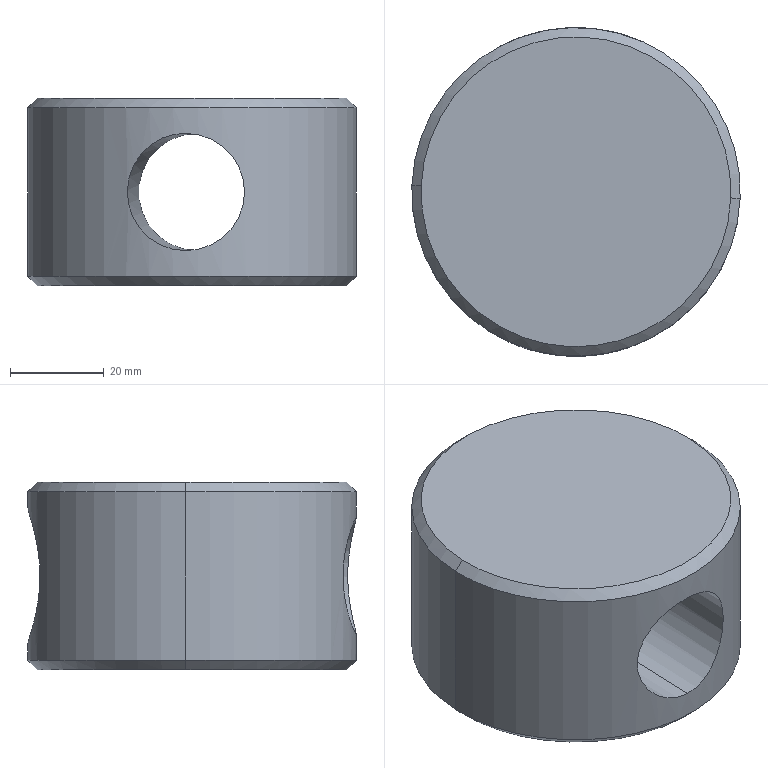Component | SolidWorks | Part3-1 | 1 solid | 13 faces | box 70 x 70 x 40 mm | volume 118313 mm3 | cylinder 6 | cone 4 | plane 3 | commonest cylinder face diameters 29 x2 25 x2 70 x2
build123d program:
from build123d import *

# Parameters (mm, degrees)
BOSS_EXTRUDE1_DEPTH   = 20
HOLE1_D               = 25
HOLE1_DEPTH           = 93.98
HOLE1_ON_FACE_2_D     = 25
HOLE1_ON_FACE_2_DEPTH = 93.98
HOLE2_D               = 29
HOLE2_DEPTH           = 7
CHAMFER1_SIZE         = 2


with BuildPart() as part:
    # Sketch1 → Boss-Extrude1 (new, symmetric)
    with BuildSketch(Plane.XY):
        with BuildLine():
            ThreePointArc((35, 0), (29.432, 18.941), (14.5, 31.855))
            Line((14.5, 31.855), (14.5, 24.855))
            Line((14.5, 24.855), (12.5, 24.855))
            Line((12.5, 24.855), (12.5, -32.692))
            ThreePointArc((12.5, -32.692), (28.831, -19.843), (35, 0))
        make_face()
        with BuildLine():
            Line((0, 24.855), (0, 35))
            ThreePointArc((0, 35), (-35, 0), (0, -35))
            Line((0, -35), (0, 24.855))
        make_face()
        with BuildLine():
            Line((12.5, 24.855), (0, 24.855))
            Line((0, 24.855), (0, -35))
            ThreePointArc((0, -35), (6.356, -34.418), (12.5, -32.692))
            Line((12.5, -32.692), (12.5, 24.855))
        make_face()
        with BuildLine():
            ThreePointArc((14.5, 31.855), (7.419, 34.205), (0, 35))
            Line((0, 35), (0, 24.855))
            Line((0, 24.855), (12.5, 24.855))
            Line((12.5, 24.855), (14.5, 24.855))
            Line((14.5, 24.855), (14.5, 31.855))
        make_face()
    extrude(amount=BOSS_EXTRUDE1_DEPTH, both=True)

    # Hole1
    with Locations(Plane(origin=(0, 35, 0), x_dir=(1, 0, 0), z_dir=(0, 1, 0))):
        with Locations((0, 0)):
            Hole(HOLE1_D / 2, depth=HOLE1_DEPTH)

    # Hole1 on face 2
    with Locations(Plane(origin=(0, 41.874, 0), x_dir=(1, 0, 0), z_dir=(0, 1, 0))):
        with Locations((0, 0)):
            Hole(HOLE1_ON_FACE_2_D / 2, depth=HOLE1_ON_FACE_2_DEPTH)

    # Hole2
    with Locations(Plane(origin=(0, 35, 0), x_dir=(1, 0, 0), z_dir=(0, 1, 0))):
        with Locations((0, 0)):
            Hole(HOLE2_D / 2, depth=HOLE2_DEPTH)

    # Chamfer1
    chamfer1_edges = [part.edges().sort_by_distance(p)[0] for p in [
        (29.432, 18.941, -20),
        (29.432, 18.941, 20),
    ]]
    chamfer(chamfer1_edges, length=CHAMFER1_SIZE)


solid = part.part

# Placed as in the assembly
solid = solid.moved(Location((-80.719, 26.515, 130), (0.000125, 0, -2.258)))
STEP:
#1=COLOUR_RGB('',0.7922,0.8196,0.9333);
#2=FILL_AREA_STYLE_COLOUR('',#1);
#3=FILL_AREA_STYLE('',(#2));
#4=SURFACE_STYLE_FILL_AREA(#3);
#5=SURFACE_SIDE_STYLE('',(#4));
#6=SURFACE_STYLE_USAGE(.BOTH.,#5);
#7=PRESENTATION_STYLE_ASSIGNMENT((#6));
#8=CARTESIAN_POINT('',(-1.88,0.9927,5.906));
#9=VERTEX_POINT('',#8);
#10=CARTESIAN_POINT('',(-4.476,1.095,5.906));
#11=VERTEX_POINT('',#10);
#12=CARTESIAN_POINT('',(-3.178,1.044,5.906));
#13=DIRECTION('',(0.,0.,1.));
#14=DIRECTION('',(0.9992,-0.03939,0.));
#15=AXIS2_PLACEMENT_3D('',#12,#13,#14);
#16=CIRCLE('',#15,1.299);
#17=EDGE_CURVE('',#9,#11,#16,.T.);
#18=ORIENTED_EDGE('',*,*,#17,.F.);
#19=CARTESIAN_POINT('',(-1.801,0.9896,5.827));
#20=VERTEX_POINT('',#19);
#21=CARTESIAN_POINT('',(-1.88,0.9927,5.906));
#22=DIRECTION('',(0.7066,-0.02785,-0.7071));
#23=VECTOR('',#22,39.37);
#24=LINE('',#21,#23);
#25=EDGE_CURVE('',#9,#20,#24,.T.);
#26=ORIENTED_EDGE('',*,*,#25,.T.);
#27=CARTESIAN_POINT('',(-4.555,1.098,5.827));
#28=VERTEX_POINT('',#27);
#29=CARTESIAN_POINT('',(-3.178,1.044,5.827));
#30=DIRECTION('',(-0.,-0.,-1.));
#31=DIRECTION('',(0.9992,-0.03939,0.));
#32=AXIS2_PLACEMENT_3D('',#29,#30,#31);
#33=CIRCLE('',#32,1.378);
#34=EDGE_CURVE('',#28,#20,#33,.T.);
#35=ORIENTED_EDGE('',*,*,#34,.F.);
#36=CARTESIAN_POINT('',(-4.476,1.095,5.906));
#37=DIRECTION('',(-0.7066,0.02785,-0.7071));
#38=VECTOR('',#37,39.37);
#39=LINE('',#36,#38);
#40=EDGE_CURVE('',#11,#28,#39,.T.);
#41=ORIENTED_EDGE('',*,*,#40,.F.);
#42=EDGE_LOOP('',(#18,#26,#35,#41));
#43=FACE_OUTER_BOUND('',#42,.T.);
#44=CARTESIAN_POINT('',(-3.178,1.044,5.906));
#45=DIRECTION('',(-0.,-0.,-1.));
#46=DIRECTION('',(-0.9992,0.03939,0.));
#47=AXIS2_PLACEMENT_3D('',#44,#45,#46);
#48=CONICAL_SURFACE('',#47,1.299,0.7854);
#49=ADVANCED_FACE('',(#43),#48,.T.);
#50=CARTESIAN_POINT('',(-4.476,1.095,4.331));
#51=VERTEX_POINT('',#50);
#52=CARTESIAN_POINT('',(-1.88,0.9927,4.331));
#53=VERTEX_POINT('',#52);
#54=CARTESIAN_POINT('',(-3.178,1.044,4.331));
#55=DIRECTION('',(-0.,-0.,-1.));
#56=DIRECTION('',(0.9992,-0.03939,0.));
#57=AXIS2_PLACEMENT_3D('',#54,#55,#56);
#58=CIRCLE('',#57,1.299);
#59=EDGE_CURVE('',#51,#53,#58,.T.);
#60=ORIENTED_EDGE('',*,*,#59,.F.);
#61=CARTESIAN_POINT('',(-4.555,1.098,4.409));
#62=VERTEX_POINT('',#61);
#63=CARTESIAN_POINT('',(-4.555,1.098,4.409));
#64=DIRECTION('',(-0.7066,0.02785,0.7071));
#65=VECTOR('',#64,39.37);
#66=LINE('',#63,#65);
#67=EDGE_CURVE('',#51,#62,#66,.T.);
#68=ORIENTED_EDGE('',*,*,#67,.T.);
#69=CARTESIAN_POINT('',(-1.801,0.9896,4.409));
#70=VERTEX_POINT('',#69);
#71=CARTESIAN_POINT('',(-3.178,1.044,4.409));
#72=DIRECTION('',(0.,0.,1.));
#73=DIRECTION('',(0.9992,-0.03939,0.));
#74=AXIS2_PLACEMENT_3D('',#71,#72,#73);
#75=CIRCLE('',#74,1.378);
#76=EDGE_CURVE('',#70,#62,#75,.T.);
#77=ORIENTED_EDGE('',*,*,#76,.F.);
#78=CARTESIAN_POINT('',(-1.801,0.9896,4.409));
#79=DIRECTION('',(0.7066,-0.02785,0.7071));
#80=VECTOR('',#79,39.37);
#81=LINE('',#78,#80);
#82=EDGE_CURVE('',#53,#70,#81,.T.);
#83=ORIENTED_EDGE('',*,*,#82,.F.);
#84=EDGE_LOOP('',(#60,#68,#77,#83));
#85=FACE_OUTER_BOUND('',#84,.T.);
#86=CARTESIAN_POINT('',(-3.178,1.044,4.409));
#87=DIRECTION('',(0.,0.,1.));
#88=DIRECTION('',(0.9992,-0.03939,0.));
#89=AXIS2_PLACEMENT_3D('',#86,#87,#88);
#90=CONICAL_SURFACE('',#89,1.378,0.7854);
#91=ADVANCED_FACE('',(#85),#90,.T.);
#92=CARTESIAN_POINT('',(-3.134,2.145,4.547));
#93=VERTEX_POINT('',#92);
#94=CARTESIAN_POINT('',(-3.134,2.145,5.689));
#95=VERTEX_POINT('',#94);
#96=CARTESIAN_POINT('',(-3.134,2.145,5.118));
#97=DIRECTION('',(0.03939,0.9992,-0.));
#98=DIRECTION('',(0.,0.,1.));
#99=AXIS2_PLACEMENT_3D('',#96,#97,#98);
#100=CIRCLE('',#99,0.5709);
#101=EDGE_CURVE('',#93,#95,#100,.T.);
#102=ORIENTED_EDGE('',*,*,#101,.F.);
#103=CARTESIAN_POINT('',(-3.124,2.421,4.547));
#104=VERTEX_POINT('',#103);
#105=CARTESIAN_POINT('',(-3.124,2.421,4.547));
#106=DIRECTION('',(0.03939,0.9992,-0.));
#107=VECTOR('',#106,39.37);
#108=LINE('',#105,#107);
#109=EDGE_CURVE('',#93,#104,#108,.T.);
#110=ORIENTED_EDGE('',*,*,#109,.T.);
#111=CARTESIAN_POINT('',(-3.124,2.421,5.689));
#112=VERTEX_POINT('',#111);
#113=CARTESIAN_POINT('',(-3.124,2.421,5.689));
#114=CARTESIAN_POINT('',(-3.162,2.422,5.689));
#115=CARTESIAN_POINT('',(-3.199,2.422,5.685));
#116=CARTESIAN_POINT('',(-3.255,2.42,5.674));
#117=CARTESIAN_POINT('',(-3.273,2.419,5.669));
#118=CARTESIAN_POINT('',(-3.309,2.416,5.658));
#119=CARTESIAN_POINT('',(-3.327,2.414,5.652));
#120=CARTESIAN_POINT('',(-3.379,2.408,5.63));
#121=CARTESIAN_POINT('',(-3.412,2.402,5.613));
#122=CARTESIAN_POINT('',(-3.459,2.393,5.582));
#123=CARTESIAN_POINT('',(-3.474,2.39,5.57));
#124=CARTESIAN_POINT('',(-3.503,2.383,5.547));
#125=CARTESIAN_POINT('',(-3.516,2.38,5.535));
#126=CARTESIAN_POINT('',(-3.543,2.373,5.508));
#127=CARTESIAN_POINT('',(-3.555,2.369,5.495));
#128=CARTESIAN_POINT('',(-3.579,2.362,5.466));
#129=CARTESIAN_POINT('',(-3.59,2.359,5.451));
#130=CARTESIAN_POINT('',(-3.622,2.349,5.405));
#131=CARTESIAN_POINT('',(-3.64,2.342,5.372));
#132=CARTESIAN_POINT('',(-3.661,2.334,5.321));
#133=CARTESIAN_POINT('',(-3.668,2.332,5.303));
#134=CARTESIAN_POINT('',(-3.679,2.327,5.267));
#135=CARTESIAN_POINT('',(-3.684,2.326,5.249));
#136=CARTESIAN_POINT('',(-3.695,2.321,5.194));
#137=CARTESIAN_POINT('',(-3.699,2.32,5.156));
#138=CARTESIAN_POINT('',(-3.699,2.32,5.1));
#139=CARTESIAN_POINT('',(-3.698,2.32,5.081));
#140=CARTESIAN_POINT('',(-3.694,2.321,5.043));
#141=CARTESIAN_POINT('',(-3.691,2.323,5.024));
#142=CARTESIAN_POINT('',(-3.684,2.326,4.987));
#143=CARTESIAN_POINT('',(-3.679,2.327,4.969));
#144=CARTESIAN_POINT('',(-3.668,2.332,4.933));
#145=CARTESIAN_POINT('',(-3.662,2.334,4.916));
#146=CARTESIAN_POINT('',(-3.639,2.342,4.863));
#147=CARTESIAN_POINT('',(-3.622,2.349,4.831));
#148=CARTESIAN_POINT('',(-3.59,2.359,4.785));
#149=CARTESIAN_POINT('',(-3.579,2.362,4.77));
#150=CARTESIAN_POINT('',(-3.555,2.369,4.741));
#151=CARTESIAN_POINT('',(-3.542,2.373,4.727));
#152=CARTESIAN_POINT('',(-3.503,2.383,4.688));
#153=CARTESIAN_POINT('',(-3.474,2.39,4.665));
#154=CARTESIAN_POINT('',(-3.427,2.399,4.634));
#155=CARTESIAN_POINT('',(-3.411,2.402,4.624));
#156=CARTESIAN_POINT('',(-3.378,2.407,4.606));
#157=CARTESIAN_POINT('',(-3.361,2.41,4.598));
#158=CARTESIAN_POINT('',(-3.309,2.416,4.577));
#159=CARTESIAN_POINT('',(-3.274,2.419,4.566));
#160=CARTESIAN_POINT('',(-3.218,2.421,4.555));
#161=CARTESIAN_POINT('',(-3.199,2.422,4.552));
#162=CARTESIAN_POINT('',(-3.161,2.422,4.548));
#163=CARTESIAN_POINT('',(-3.142,2.422,4.547));
#164=CARTESIAN_POINT('',(-3.124,2.421,4.547));
#165=B_SPLINE_CURVE_WITH_KNOTS('',3,(#113,#114,#115,#116,#117,#118,#119,#120,#121,#122,#123,#124,#125,#126,#127,#128,#129,#130,#131,#132,#133,#134,#135,#136,#137,#138,#139,#140,#141,#142,#143,#144,#145,#146,#147,#148,#149,#150,#151,#152,#153,#154,#155,#156,#157,#158,#159,#160,#161,#162,#163,#164),.UNSPECIFIED.,.F.,.F.,(4,2,2,2,2,2,2,2,2,2,2,2,2,2,2,2,2,2,2,2,2,2,2,2,2,4),(0.,0.002866,0.004299,0.005732,0.008598,0.01003,0.01146,0.0129,0.01433,0.0172,0.01863,0.02006,0.02293,0.02436,0.02579,0.02723,0.02866,0.03153,0.03296,0.03439,0.03726,0.03869,0.04012,0.04299,0.04442,0.04586),.UNSPECIFIED.);
#166=EDGE_CURVE('',#112,#104,#165,.T.);
#167=ORIENTED_EDGE('',*,*,#166,.F.);
#168=CARTESIAN_POINT('',(-3.124,2.421,5.689));
#169=DIRECTION('',(0.03939,0.9992,-0.));
#170=VECTOR('',#169,39.37);
#171=LINE('',#168,#170);
#172=EDGE_CURVE('',#95,#112,#171,.T.);
#173=ORIENTED_EDGE('',*,*,#172,.F.);
#174=EDGE_LOOP('',(#102,#110,#167,#173));
#175=FACE_OUTER_BOUND('',#174,.T.);
#176=CARTESIAN_POINT('',(-3.124,2.421,5.118));
#177=DIRECTION('',(0.03939,0.9992,-0.));
#178=DIRECTION('',(0.,0.,1.));
#179=AXIS2_PLACEMENT_3D('',#176,#177,#178);
#180=CYLINDRICAL_SURFACE('',#179,0.5709);
#181=ADVANCED_FACE('',(#175),#180,.F.);
#182=CARTESIAN_POINT('',(-3.232,-0.333,4.626));
#183=VERTEX_POINT('',#182);
#184=CARTESIAN_POINT('',(-3.232,-0.333,5.61));
#185=VERTEX_POINT('',#184);
#186=CARTESIAN_POINT('',(-3.232,-0.333,4.626));
#187=CARTESIAN_POINT('',(-3.248,-0.3324,4.626));
#188=CARTESIAN_POINT('',(-3.264,-0.3314,4.627));
#189=CARTESIAN_POINT('',(-3.297,-0.329,4.63));
#190=CARTESIAN_POINT('',(-3.313,-0.3275,4.632));
#191=CARTESIAN_POINT('',(-3.361,-0.3223,4.642));
#192=CARTESIAN_POINT('',(-3.391,-0.3178,4.651));
#193=CARTESIAN_POINT('',(-3.436,-0.3099,4.67));
#194=CARTESIAN_POINT('',(-3.45,-0.307,4.677));
#195=CARTESIAN_POINT('',(-3.478,-0.301,4.692));
#196=CARTESIAN_POINT('',(-3.492,-0.2979,4.701));
#197=CARTESIAN_POINT('',(-3.531,-0.2882,4.727));
#198=CARTESIAN_POINT('',(-3.556,-0.2814,4.748));
#199=CARTESIAN_POINT('',(-3.59,-0.2712,4.782));
#200=CARTESIAN_POINT('',(-3.6,-0.2678,4.794));
#201=CARTESIAN_POINT('',(-3.62,-0.2612,4.818));
#202=CARTESIAN_POINT('',(-3.63,-0.258,4.831));
#203=CARTESIAN_POINT('',(-3.647,-0.2518,4.858));
#204=CARTESIAN_POINT('',(-3.655,-0.2488,4.871));
#205=CARTESIAN_POINT('',(-3.67,-0.2432,4.899));
#206=CARTESIAN_POINT('',(-3.677,-0.2405,4.914));
#207=CARTESIAN_POINT('',(-3.695,-0.2333,4.959));
#208=CARTESIAN_POINT('',(-3.705,-0.2294,4.99));
#209=CARTESIAN_POINT('',(-3.714,-0.2255,5.037));
#210=CARTESIAN_POINT('',(-3.716,-0.2245,5.053));
#211=CARTESIAN_POINT('',(-3.72,-0.2231,5.086));
#212=CARTESIAN_POINT('',(-3.72,-0.2228,5.102));
#213=CARTESIAN_POINT('',(-3.72,-0.2228,5.151));
#214=CARTESIAN_POINT('',(-3.717,-0.2242,5.183));
#215=CARTESIAN_POINT('',(-3.708,-0.2281,5.231));
#216=CARTESIAN_POINT('',(-3.704,-0.2298,5.247));
#217=CARTESIAN_POINT('',(-3.695,-0.2336,5.277));
#218=CARTESIAN_POINT('',(-3.689,-0.2357,5.293));
#219=CARTESIAN_POINT('',(-3.677,-0.2405,5.322));
#220=CARTESIAN_POINT('',(-3.67,-0.2432,5.337));
#221=CARTESIAN_POINT('',(-3.655,-0.2488,5.365));
#222=CARTESIAN_POINT('',(-3.647,-0.2518,5.379));
#223=CARTESIAN_POINT('',(-3.62,-0.2612,5.419));
#224=CARTESIAN_POINT('',(-3.6,-0.2679,5.444));
#225=CARTESIAN_POINT('',(-3.556,-0.2814,5.489));
#226=CARTESIAN_POINT('',(-3.531,-0.2883,5.509));
#227=CARTESIAN_POINT('',(-3.478,-0.3012,5.545));
#228=CARTESIAN_POINT('',(-3.45,-0.3072,5.56));
#229=CARTESIAN_POINT('',(-3.406,-0.3151,5.579));
#230=CARTESIAN_POINT('',(-3.391,-0.3176,5.584));
#231=CARTESIAN_POINT('',(-3.36,-0.3221,5.594));
#232=CARTESIAN_POINT('',(-3.344,-0.3241,5.598));
#233=CARTESIAN_POINT('',(-3.297,-0.3293,5.607));
#234=CARTESIAN_POINT('',(-3.265,-0.3317,5.61));
#235=CARTESIAN_POINT('',(-3.232,-0.333,5.61));
#236=B_SPLINE_CURVE_WITH_KNOTS('',3,(#186,#187,#188,#189,#190,#191,#192,#193,#194,#195,#196,#197,#198,#199,#200,#201,#202,#203,#204,#205,#206,#207,#208,#209,#210,#211,#212,#213,#214,#215,#216,#217,#218,#219,#220,#221,#222,#223,#224,#225,#226,#227,#228,#229,#230,#231,#232,#233,#234,#235),.UNSPECIFIED.,.F.,.F.,(4,2,2,2,2,2,2,2,2,2,2,2,2,2,2,2,2,2,2,2,2,2,2,2,4),(0.03941,0.04064,0.04187,0.04433,0.04557,0.0468,0.04926,0.05049,0.05172,0.05295,0.05418,0.05665,0.05788,0.05911,0.06157,0.0628,0.06403,0.06526,0.0665,0.06896,0.07142,0.07388,0.07511,0.07635,0.07881),.UNSPECIFIED.);
#237=EDGE_CURVE('',#183,#185,#236,.T.);
#238=ORIENTED_EDGE('',*,*,#237,.F.);
#239=CARTESIAN_POINT('',(-3.134,2.145,4.626));
#240=VERTEX_POINT('',#239);
#241=CARTESIAN_POINT('',(-3.124,2.421,4.626));
#242=DIRECTION('',(0.03939,0.9992,-0.));
#243=VECTOR('',#242,39.37);
#244=LINE('',#241,#243);
#245=EDGE_CURVE('',#183,#240,#244,.T.);
#246=ORIENTED_EDGE('',*,*,#245,.T.);
#247=CARTESIAN_POINT('',(-3.134,2.145,5.61));
#248=VERTEX_POINT('',#247);
#249=CARTESIAN_POINT('',(-3.134,2.145,5.118));
#250=DIRECTION('',(0.03939,0.9992,-0.));
#251=DIRECTION('',(-0.,0.,-1.));
#252=AXIS2_PLACEMENT_3D('',#249,#250,#251);
#253=CIRCLE('',#252,0.4921);
#254=EDGE_CURVE('',#240,#248,#253,.T.);
#255=ORIENTED_EDGE('',*,*,#254,.T.);
#256=CARTESIAN_POINT('',(-3.124,2.421,5.61));
#257=DIRECTION('',(0.03939,0.9992,-0.));
#258=VECTOR('',#257,39.37);
#259=LINE('',#256,#258);
#260=EDGE_CURVE('',#185,#248,#259,.T.);
#261=ORIENTED_EDGE('',*,*,#260,.F.);
#262=EDGE_LOOP('',(#238,#246,#255,#261));
#263=FACE_OUTER_BOUND('',#262,.T.);
#264=CARTESIAN_POINT('',(-3.124,2.421,5.118));
#265=DIRECTION('',(0.03939,0.9992,-0.));
#266=DIRECTION('',(0.,0.,1.));
#267=AXIS2_PLACEMENT_3D('',#264,#265,#266);
#268=CYLINDRICAL_SURFACE('',#267,0.4921);
#269=ADVANCED_FACE('',(#263),#268,.F.);
#270=ORIENTED_EDGE('',*,*,#166,.T.);
#271=CARTESIAN_POINT('',(-3.124,2.421,4.547));
#272=CARTESIAN_POINT('',(-3.105,2.42,4.547));
#273=CARTESIAN_POINT('',(-3.086,2.419,4.548));
#274=CARTESIAN_POINT('',(-3.048,2.416,4.552));
#275=CARTESIAN_POINT('',(-3.03,2.414,4.555));
#276=CARTESIAN_POINT('',(-2.974,2.407,4.566));
#277=CARTESIAN_POINT('',(-2.939,2.401,4.577));
#278=CARTESIAN_POINT('',(-2.887,2.391,4.599));
#279=CARTESIAN_POINT('',(-2.87,2.387,4.607));
#280=CARTESIAN_POINT('',(-2.838,2.379,4.624));
#281=CARTESIAN_POINT('',(-2.822,2.375,4.634));
#282=CARTESIAN_POINT('',(-2.792,2.367,4.655));
#283=CARTESIAN_POINT('',(-2.777,2.362,4.666));
#284=CARTESIAN_POINT('',(-2.749,2.353,4.689));
#285=CARTESIAN_POINT('',(-2.735,2.349,4.702));
#286=CARTESIAN_POINT('',(-2.696,2.335,4.741));
#287=CARTESIAN_POINT('',(-2.673,2.326,4.77));
#288=CARTESIAN_POINT('',(-2.643,2.314,4.815));
#289=CARTESIAN_POINT('',(-2.634,2.31,4.831));
#290=CARTESIAN_POINT('',(-2.616,2.302,4.864));
#291=CARTESIAN_POINT('',(-2.608,2.299,4.881));
#292=CARTESIAN_POINT('',(-2.587,2.289,4.933));
#293=CARTESIAN_POINT('',(-2.576,2.284,4.968));
#294=CARTESIAN_POINT('',(-2.566,2.278,5.024));
#295=CARTESIAN_POINT('',(-2.563,2.277,5.042));
#296=CARTESIAN_POINT('',(-2.559,2.275,5.08));
#297=CARTESIAN_POINT('',(-2.558,2.275,5.099));
#298=CARTESIAN_POINT('',(-2.558,2.275,5.156));
#299=CARTESIAN_POINT('',(-2.562,2.276,5.193));
#300=CARTESIAN_POINT('',(-2.576,2.284,5.268));
#301=CARTESIAN_POINT('',(-2.587,2.289,5.303));
#302=CARTESIAN_POINT('',(-2.608,2.299,5.355));
#303=CARTESIAN_POINT('',(-2.616,2.302,5.372));
#304=CARTESIAN_POINT('',(-2.634,2.31,5.405));
#305=CARTESIAN_POINT('',(-2.643,2.314,5.421));
#306=CARTESIAN_POINT('',(-2.674,2.326,5.467));
#307=CARTESIAN_POINT('',(-2.697,2.335,5.495));
#308=CARTESIAN_POINT('',(-2.735,2.349,5.535));
#309=CARTESIAN_POINT('',(-2.749,2.353,5.547));
#310=CARTESIAN_POINT('',(-2.777,2.362,5.571));
#311=CARTESIAN_POINT('',(-2.792,2.367,5.582));
#312=CARTESIAN_POINT('',(-2.837,2.379,5.613));
#313=CARTESIAN_POINT('',(-2.87,2.387,5.63));
#314=CARTESIAN_POINT('',(-2.939,2.401,5.659));
#315=CARTESIAN_POINT('',(-2.975,2.407,5.67));
#316=CARTESIAN_POINT('',(-3.029,2.414,5.681));
#317=CARTESIAN_POINT('',(-3.048,2.416,5.684));
#318=CARTESIAN_POINT('',(-3.085,2.419,5.688));
#319=CARTESIAN_POINT('',(-3.105,2.42,5.689));
#320=CARTESIAN_POINT('',(-3.124,2.421,5.689));
#321=B_SPLINE_CURVE_WITH_KNOTS('',3,(#271,#272,#273,#274,#275,#276,#277,#278,#279,#280,#281,#282,#283,#284,#285,#286,#287,#288,#289,#290,#291,#292,#293,#294,#295,#296,#297,#298,#299,#300,#301,#302,#303,#304,#305,#306,#307,#308,#309,#310,#311,#312,#313,#314,#315,#316,#317,#318,#319,#320),.UNSPECIFIED.,.F.,.F.,(4,2,2,2,2,2,2,2,2,2,2,2,2,2,2,2,2,2,2,2,2,2,2,2,4),(0.04586,0.04729,0.04872,0.05158,0.05302,0.05445,0.05588,0.05731,0.06018,0.06161,0.06304,0.0659,0.06733,0.06877,0.07163,0.07449,0.07593,0.07736,0.08022,0.08165,0.08309,0.08595,0.08881,0.09025,0.09168),.UNSPECIFIED.);
#322=EDGE_CURVE('',#104,#112,#321,.T.);
#323=ORIENTED_EDGE('',*,*,#322,.T.);
#324=EDGE_LOOP('',(#270,#323));
#325=FACE_BOUND('',#324,.T.);
#326=ORIENTED_EDGE('',*,*,#34,.T.);
#327=CARTESIAN_POINT('',(-1.801,0.9896,5.906));
#328=DIRECTION('',(-0.,-0.,-1.));
#329=VECTOR('',#328,39.37);
#330=LINE('',#327,#329);
#331=EDGE_CURVE('',#20,#70,#330,.T.);
#332=ORIENTED_EDGE('',*,*,#331,.T.);
#333=ORIENTED_EDGE('',*,*,#76,.T.);
#334=CARTESIAN_POINT('',(-4.555,1.098,5.906));
#335=DIRECTION('',(-0.,-0.,-1.));
#336=VECTOR('',#335,39.37);
#337=LINE('',#334,#336);
#338=EDGE_CURVE('',#28,#62,#337,.T.);
#339=ORIENTED_EDGE('',*,*,#338,.F.);
#340=EDGE_LOOP('',(#326,#332,#333,#339));
#341=FACE_OUTER_BOUND('',#340,.T.);
#342=CARTESIAN_POINT('',(-3.178,1.044,5.906));
#343=DIRECTION('',(-0.,-0.,-1.));
#344=DIRECTION('',(-0.9992,0.03939,0.));
#345=AXIS2_PLACEMENT_3D('',#342,#343,#344);
#346=CYLINDRICAL_SURFACE('',#345,1.378);
#347=ADVANCED_FACE('',(#325,#341),#346,.T.);
#348=ORIENTED_EDGE('',*,*,#331,.F.);
#349=CARTESIAN_POINT('',(-3.178,1.044,5.827));
#350=DIRECTION('',(-0.,-0.,-1.));
#351=DIRECTION('',(0.9992,-0.03939,0.));
#352=AXIS2_PLACEMENT_3D('',#349,#350,#351);
#353=CIRCLE('',#352,1.378);
#354=EDGE_CURVE('',#20,#28,#353,.T.);
#355=ORIENTED_EDGE('',*,*,#354,.T.);
#356=ORIENTED_EDGE('',*,*,#338,.T.);
#357=CARTESIAN_POINT('',(-3.178,1.044,4.409));
#358=DIRECTION('',(0.,0.,1.));
#359=DIRECTION('',(0.9992,-0.03939,0.));
#360=AXIS2_PLACEMENT_3D('',#357,#358,#359);
#361=CIRCLE('',#360,1.378);
#362=EDGE_CURVE('',#62,#70,#361,.T.);
#363=ORIENTED_EDGE('',*,*,#362,.T.);
#364=EDGE_LOOP('',(#348,#355,#356,#363));
#365=FACE_OUTER_BOUND('',#364,.T.);
#366=CARTESIAN_POINT('',(-3.232,-0.333,5.61));
#367=CARTESIAN_POINT('',(-3.199,-0.3343,5.61));
#368=CARTESIAN_POINT('',(-3.167,-0.3344,5.607));
#369=CARTESIAN_POINT('',(-3.12,-0.3329,5.597));
#370=CARTESIAN_POINT('',(-3.104,-0.3322,5.594));
#371=CARTESIAN_POINT('',(-3.073,-0.3301,5.584));
#372=CARTESIAN_POINT('',(-3.057,-0.3289,5.579));
#373=CARTESIAN_POINT('',(-3.012,-0.3244,5.56));
#374=CARTESIAN_POINT('',(-2.984,-0.3206,5.545));
#375=CARTESIAN_POINT('',(-2.944,-0.3141,5.518));
#376=CARTESIAN_POINT('',(-2.931,-0.3118,5.508));
#377=CARTESIAN_POINT('',(-2.906,-0.307,5.488));
#378=CARTESIAN_POINT('',(-2.894,-0.3045,5.477));
#379=CARTESIAN_POINT('',(-2.86,-0.2971,5.443));
#380=CARTESIAN_POINT('',(-2.839,-0.292,5.419));
#381=CARTESIAN_POINT('',(-2.803,-0.2822,5.365));
#382=CARTESIAN_POINT('',(-2.788,-0.2777,5.337));
#383=CARTESIAN_POINT('',(-2.769,-0.272,5.293));
#384=CARTESIAN_POINT('',(-2.763,-0.2703,5.277));
#385=CARTESIAN_POINT('',(-2.754,-0.2672,5.247));
#386=CARTESIAN_POINT('',(-2.75,-0.2659,5.231));
#387=CARTESIAN_POINT('',(-2.74,-0.2627,5.183));
#388=CARTESIAN_POINT('',(-2.737,-0.2616,5.151));
#389=CARTESIAN_POINT('',(-2.737,-0.2616,5.102));
#390=CARTESIAN_POINT('',(-2.738,-0.2618,5.086));
#391=CARTESIAN_POINT('',(-2.741,-0.2629,5.053));
#392=CARTESIAN_POINT('',(-2.743,-0.2638,5.037));
#393=CARTESIAN_POINT('',(-2.753,-0.2669,4.99));
#394=CARTESIAN_POINT('',(-2.763,-0.27,4.959));
#395=CARTESIAN_POINT('',(-2.788,-0.2778,4.899));
#396=CARTESIAN_POINT('',(-2.803,-0.2823,4.871));
#397=CARTESIAN_POINT('',(-2.83,-0.2895,4.831));
#398=CARTESIAN_POINT('',(-2.84,-0.292,4.818));
#399=CARTESIAN_POINT('',(-2.86,-0.297,4.793));
#400=CARTESIAN_POINT('',(-2.871,-0.2996,4.781));
#401=CARTESIAN_POINT('',(-2.906,-0.3071,4.747));
#402=CARTESIAN_POINT('',(-2.93,-0.3119,4.727));
#403=CARTESIAN_POINT('',(-2.971,-0.3185,4.7));
#404=CARTESIAN_POINT('',(-2.985,-0.3205,4.692));
#405=CARTESIAN_POINT('',(-3.013,-0.3243,4.677));
#406=CARTESIAN_POINT('',(-3.028,-0.326,4.67));
#407=CARTESIAN_POINT('',(-3.072,-0.3304,4.651));
#408=CARTESIAN_POINT('',(-3.103,-0.3324,4.642));
#409=CARTESIAN_POINT('',(-3.151,-0.3339,4.632));
#410=CARTESIAN_POINT('',(-3.168,-0.3341,4.63));
#411=CARTESIAN_POINT('',(-3.2,-0.334,4.627));
#412=CARTESIAN_POINT('',(-3.216,-0.3336,4.626));
#413=CARTESIAN_POINT('',(-3.232,-0.333,4.626));
#414=B_SPLINE_CURVE_WITH_KNOTS('',3,(#366,#367,#368,#369,#370,#371,#372,#373,#374,#375,#376,#377,#378,#379,#380,#381,#382,#383,#384,#385,#386,#387,#388,#389,#390,#391,#392,#393,#394,#395,#396,#397,#398,#399,#400,#401,#402,#403,#404,#405,#406,#407,#408,#409,#410,#411,#412,#413),.UNSPECIFIED.,.F.,.F.,(4,2,2,2,2,2,2,2,2,2,2,2,2,2,2,2,2,2,2,2,2,2,2,4),(0.,0.002463,0.003695,0.004926,0.007389,0.008621,0.009852,0.01232,0.01478,0.01601,0.01724,0.0197,0.02094,0.02217,0.02463,0.02709,0.02833,0.02956,0.03202,0.03325,0.03448,0.03695,0.03818,0.03941),.UNSPECIFIED.);
#415=EDGE_CURVE('',#185,#183,#414,.T.);
#416=ORIENTED_EDGE('',*,*,#415,.T.);
#417=ORIENTED_EDGE('',*,*,#237,.T.);
#418=EDGE_LOOP('',(#416,#417));
#419=FACE_BOUND('',#418,.T.);
#420=CARTESIAN_POINT('',(-3.178,1.044,5.906));
#421=DIRECTION('',(-0.,-0.,-1.));
#422=DIRECTION('',(-0.9992,0.03939,0.));
#423=AXIS2_PLACEMENT_3D('',#420,#421,#422);
#424=CYLINDRICAL_SURFACE('',#423,1.378);
#425=ADVANCED_FACE('',(#365,#419),#424,.T.);
#426=CARTESIAN_POINT('',(-3.178,1.044,5.906));
#427=DIRECTION('',(0.,0.,1.));
#428=DIRECTION('',(0.9992,-0.03939,0.));
#429=AXIS2_PLACEMENT_3D('',#426,#427,#428);
#430=CIRCLE('',#429,1.299);
#431=EDGE_CURVE('',#11,#9,#430,.T.);
#432=ORIENTED_EDGE('',*,*,#431,.T.);
#433=ORIENTED_EDGE('',*,*,#17,.T.);
#434=EDGE_LOOP('',(#432,#433));
#435=FACE_OUTER_BOUND('',#434,.T.);
#436=CARTESIAN_POINT('',(-3.178,1.044,5.906));
#437=DIRECTION('',(0.,0.,1.));
#438=DIRECTION('',(0.9992,-0.03939,-0.));
#439=AXIS2_PLACEMENT_3D('',#436,#437,#438);
#440=PLANE('',#439);
#441=ADVANCED_FACE('',(#435),#440,.T.);
#442=CARTESIAN_POINT('',(-3.178,1.044,4.331));
#443=DIRECTION('',(-0.,-0.,-1.));
#444=DIRECTION('',(0.9992,-0.03939,0.));
#445=AXIS2_PLACEMENT_3D('',#442,#443,#444);
#446=CIRCLE('',#445,1.299);
#447=EDGE_CURVE('',#53,#51,#446,.T.);
#448=ORIENTED_EDGE('',*,*,#447,.T.);
#449=ORIENTED_EDGE('',*,*,#59,.T.);
#450=EDGE_LOOP('',(#448,#449));
#451=FACE_OUTER_BOUND('',#450,.T.);
#452=CARTESIAN_POINT('',(-3.178,1.044,4.331));
#453=DIRECTION('',(0.,0.,1.));
#454=DIRECTION('',(0.9992,-0.03939,-0.));
#455=AXIS2_PLACEMENT_3D('',#452,#453,#454);
#456=PLANE('',#455);
#457=ADVANCED_FACE('',(#451),#456,.F.);
#458=ORIENTED_EDGE('',*,*,#245,.F.);
#459=ORIENTED_EDGE('',*,*,#415,.F.);
#460=ORIENTED_EDGE('',*,*,#260,.T.);
#461=CARTESIAN_POINT('',(-3.134,2.145,5.118));
#462=DIRECTION('',(0.03939,0.9992,-0.));
#463=DIRECTION('',(0.,0.,-1.));
#464=AXIS2_PLACEMENT_3D('',#461,#462,#463);
#465=CIRCLE('',#464,0.4921);
#466=EDGE_CURVE('',#248,#240,#465,.T.);
#467=ORIENTED_EDGE('',*,*,#466,.T.);
#468=EDGE_LOOP('',(#458,#459,#460,#467));
#469=FACE_OUTER_BOUND('',#468,.T.);
#470=CARTESIAN_POINT('',(-3.124,2.421,5.118));
#471=DIRECTION('',(0.03939,0.9992,-0.));
#472=DIRECTION('',(0.,0.,1.));
#473=AXIS2_PLACEMENT_3D('',#470,#471,#472);
#474=CYLINDRICAL_SURFACE('',#473,0.4921);
#475=ADVANCED_FACE('',(#469),#474,.F.);
#476=CARTESIAN_POINT('',(-3.134,2.145,5.118));
#477=DIRECTION('',(0.03939,0.9992,-0.));
#478=DIRECTION('',(0.,0.,1.));
#479=AXIS2_PLACEMENT_3D('',#476,#477,#478);
#480=CIRCLE('',#479,0.5709);
#481=EDGE_CURVE('',#95,#93,#480,.T.);
#482=ORIENTED_EDGE('',*,*,#481,.T.);
#483=ORIENTED_EDGE('',*,*,#101,.T.);
#484=EDGE_LOOP('',(#482,#483));
#485=FACE_OUTER_BOUND('',#484,.T.);
#486=ORIENTED_EDGE('',*,*,#466,.F.);
#487=ORIENTED_EDGE('',*,*,#254,.F.);
#488=EDGE_LOOP('',(#486,#487));
#489=FACE_BOUND('',#488,.T.);
#490=CARTESIAN_POINT('',(-3.134,2.145,5.118));
#491=DIRECTION('',(-0.03939,-0.9992,0.));
#492=DIRECTION('',(-0.,-0.,-1.));
#493=AXIS2_PLACEMENT_3D('',#490,#491,#492);
#494=PLANE('',#493);
#495=ADVANCED_FACE('',(#485,#489),#494,.F.);
#496=ORIENTED_EDGE('',*,*,#109,.F.);
#497=ORIENTED_EDGE('',*,*,#481,.F.);
#498=ORIENTED_EDGE('',*,*,#172,.T.);
#499=ORIENTED_EDGE('',*,*,#322,.F.);
#500=EDGE_LOOP('',(#496,#497,#498,#499));
#501=FACE_OUTER_BOUND('',#500,.T.);
#502=CARTESIAN_POINT('',(-3.124,2.421,5.118));
#503=DIRECTION('',(0.03939,0.9992,-0.));
#504=DIRECTION('',(0.,0.,1.));
#505=AXIS2_PLACEMENT_3D('',#502,#503,#504);
#506=CYLINDRICAL_SURFACE('',#505,0.5709);
#507=ADVANCED_FACE('',(#501),#506,.F.);
#508=ORIENTED_EDGE('',*,*,#67,.F.);
#509=ORIENTED_EDGE('',*,*,#447,.F.);
#510=ORIENTED_EDGE('',*,*,#82,.T.);
#511=ORIENTED_EDGE('',*,*,#362,.F.);
#512=EDGE_LOOP('',(#508,#509,#510,#511));
#513=FACE_OUTER_BOUND('',#512,.T.);
#514=CARTESIAN_POINT('',(-3.178,1.044,4.409));
#515=DIRECTION('',(0.,0.,1.));
#516=DIRECTION('',(0.9992,-0.03939,0.));
#517=AXIS2_PLACEMENT_3D('',#514,#515,#516);
#518=CONICAL_SURFACE('',#517,1.378,0.7854);
#519=ADVANCED_FACE('',(#513),#518,.T.);
#520=ORIENTED_EDGE('',*,*,#25,.F.);
#521=ORIENTED_EDGE('',*,*,#431,.F.);
#522=ORIENTED_EDGE('',*,*,#40,.T.);
#523=ORIENTED_EDGE('',*,*,#354,.F.);
#524=EDGE_LOOP('',(#520,#521,#522,#523));
#525=FACE_OUTER_BOUND('',#524,.T.);
#526=CARTESIAN_POINT('',(-3.178,1.044,5.906));
#527=DIRECTION('',(-0.,-0.,-1.));
#528=DIRECTION('',(-0.9992,0.03939,0.));
#529=AXIS2_PLACEMENT_3D('',#526,#527,#528);
#530=CONICAL_SURFACE('',#529,1.299,0.7854);
#531=ADVANCED_FACE('',(#525),#530,.T.);
#532=CLOSED_SHELL('',(#49,#91,#181,#269,#347,#425,#441,#457,#475,#495,#507,#519,#531));
#533=MANIFOLD_SOLID_BREP('',#532);
#534=STYLED_ITEM('',(#7),#533);
#535=PRESENTATION_LAYER_ASSIGNMENT('','',(#534));
#536=(LENGTH_UNIT()NAMED_UNIT(*)SI_UNIT($,.METRE.));
#537=LENGTH_MEASURE_WITH_UNIT(LENGTH_MEASURE(0.0254),#536);
#538=DIMENSIONAL_EXPONENTS(1.,0.,0.,0.,0.,0.,0.);
#539=(CONVERSION_BASED_UNIT('',#537)LENGTH_UNIT()NAMED_UNIT(#538));
#540=UNCERTAINTY_MEASURE_WITH_UNIT(LENGTH_MEASURE(0.00001),#539,'','');
#541=(NAMED_UNIT(*)PLANE_ANGLE_UNIT()SI_UNIT($,.RADIAN.));
#542=(NAMED_UNIT(*)SI_UNIT($,.STERADIAN.)SOLID_ANGLE_UNIT());
#543=(GEOMETRIC_REPRESENTATION_CONTEXT(3)GLOBAL_UNCERTAINTY_ASSIGNED_CONTEXT((#540))GLOBAL_UNIT_ASSIGNED_CONTEXT((#539,#541,#542))REPRESENTATION_CONTEXT('',''));
#544=MECHANICAL_DESIGN_GEOMETRIC_PRESENTATION_REPRESENTATION('',(#534),#543);
#545=CARTESIAN_POINT('',(0.,0.,0.));
#546=DIRECTION('',(0.,0.,1.));
#547=DIRECTION('',(1.,0.,0.));
#548=AXIS2_PLACEMENT_3D('',#545,#546,#547);
#549=(LENGTH_UNIT()NAMED_UNIT(*)SI_UNIT($,.METRE.));
#550=LENGTH_MEASURE_WITH_UNIT(LENGTH_MEASURE(0.0254),#549);
#551=DIMENSIONAL_EXPONENTS(1.,0.,0.,0.,0.,0.,0.);
#552=(CONVERSION_BASED_UNIT('',#550)LENGTH_UNIT()NAMED_UNIT(#551));
#553=UNCERTAINTY_MEASURE_WITH_UNIT(LENGTH_MEASURE(0.00001),#552,'','');
#554=(NAMED_UNIT(*)PLANE_ANGLE_UNIT()SI_UNIT($,.RADIAN.));
#555=(NAMED_UNIT(*)SI_UNIT($,.STERADIAN.)SOLID_ANGLE_UNIT());
#556=(GEOMETRIC_REPRESENTATION_CONTEXT(3)GLOBAL_UNCERTAINTY_ASSIGNED_CONTEXT((#553))GLOBAL_UNIT_ASSIGNED_CONTEXT((#552,#554,#555))REPRESENTATION_CONTEXT('',''));
#557=ADVANCED_BREP_SHAPE_REPRESENTATION('',(#533,#548),#556);